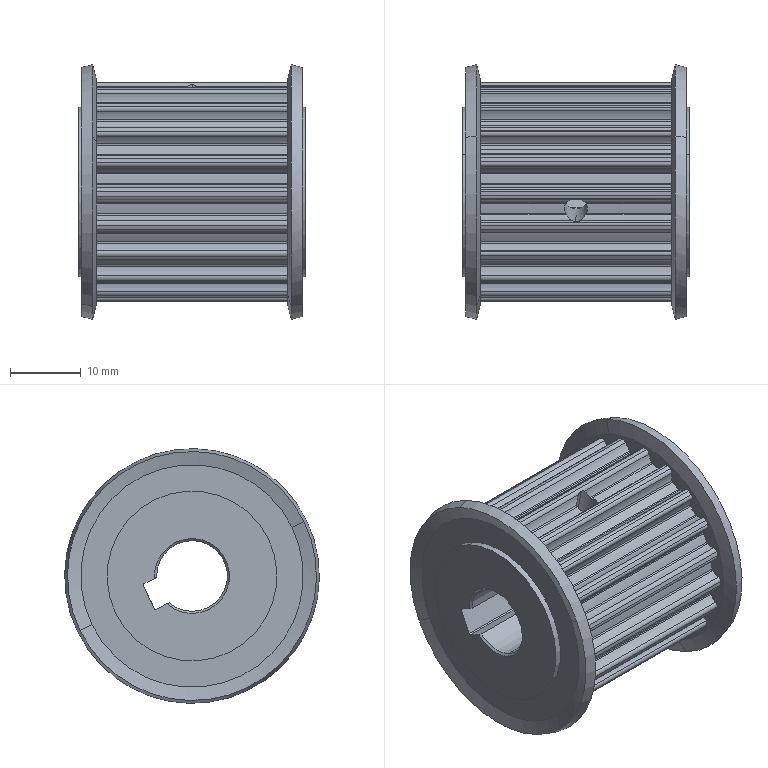Component | SolidWorks | EBJ41-S5M250-20-A-N-d10-4 | 1 solid | 231 faces | volume 18771 mm3 | cylinder 204 | cone 18 | plane 9 | commonest cylinder face diameters 1.1 x50 0.5 x50 6.55 x48 27.33 x23 30.87 x20 3.242 x4 24 x4 10 x3